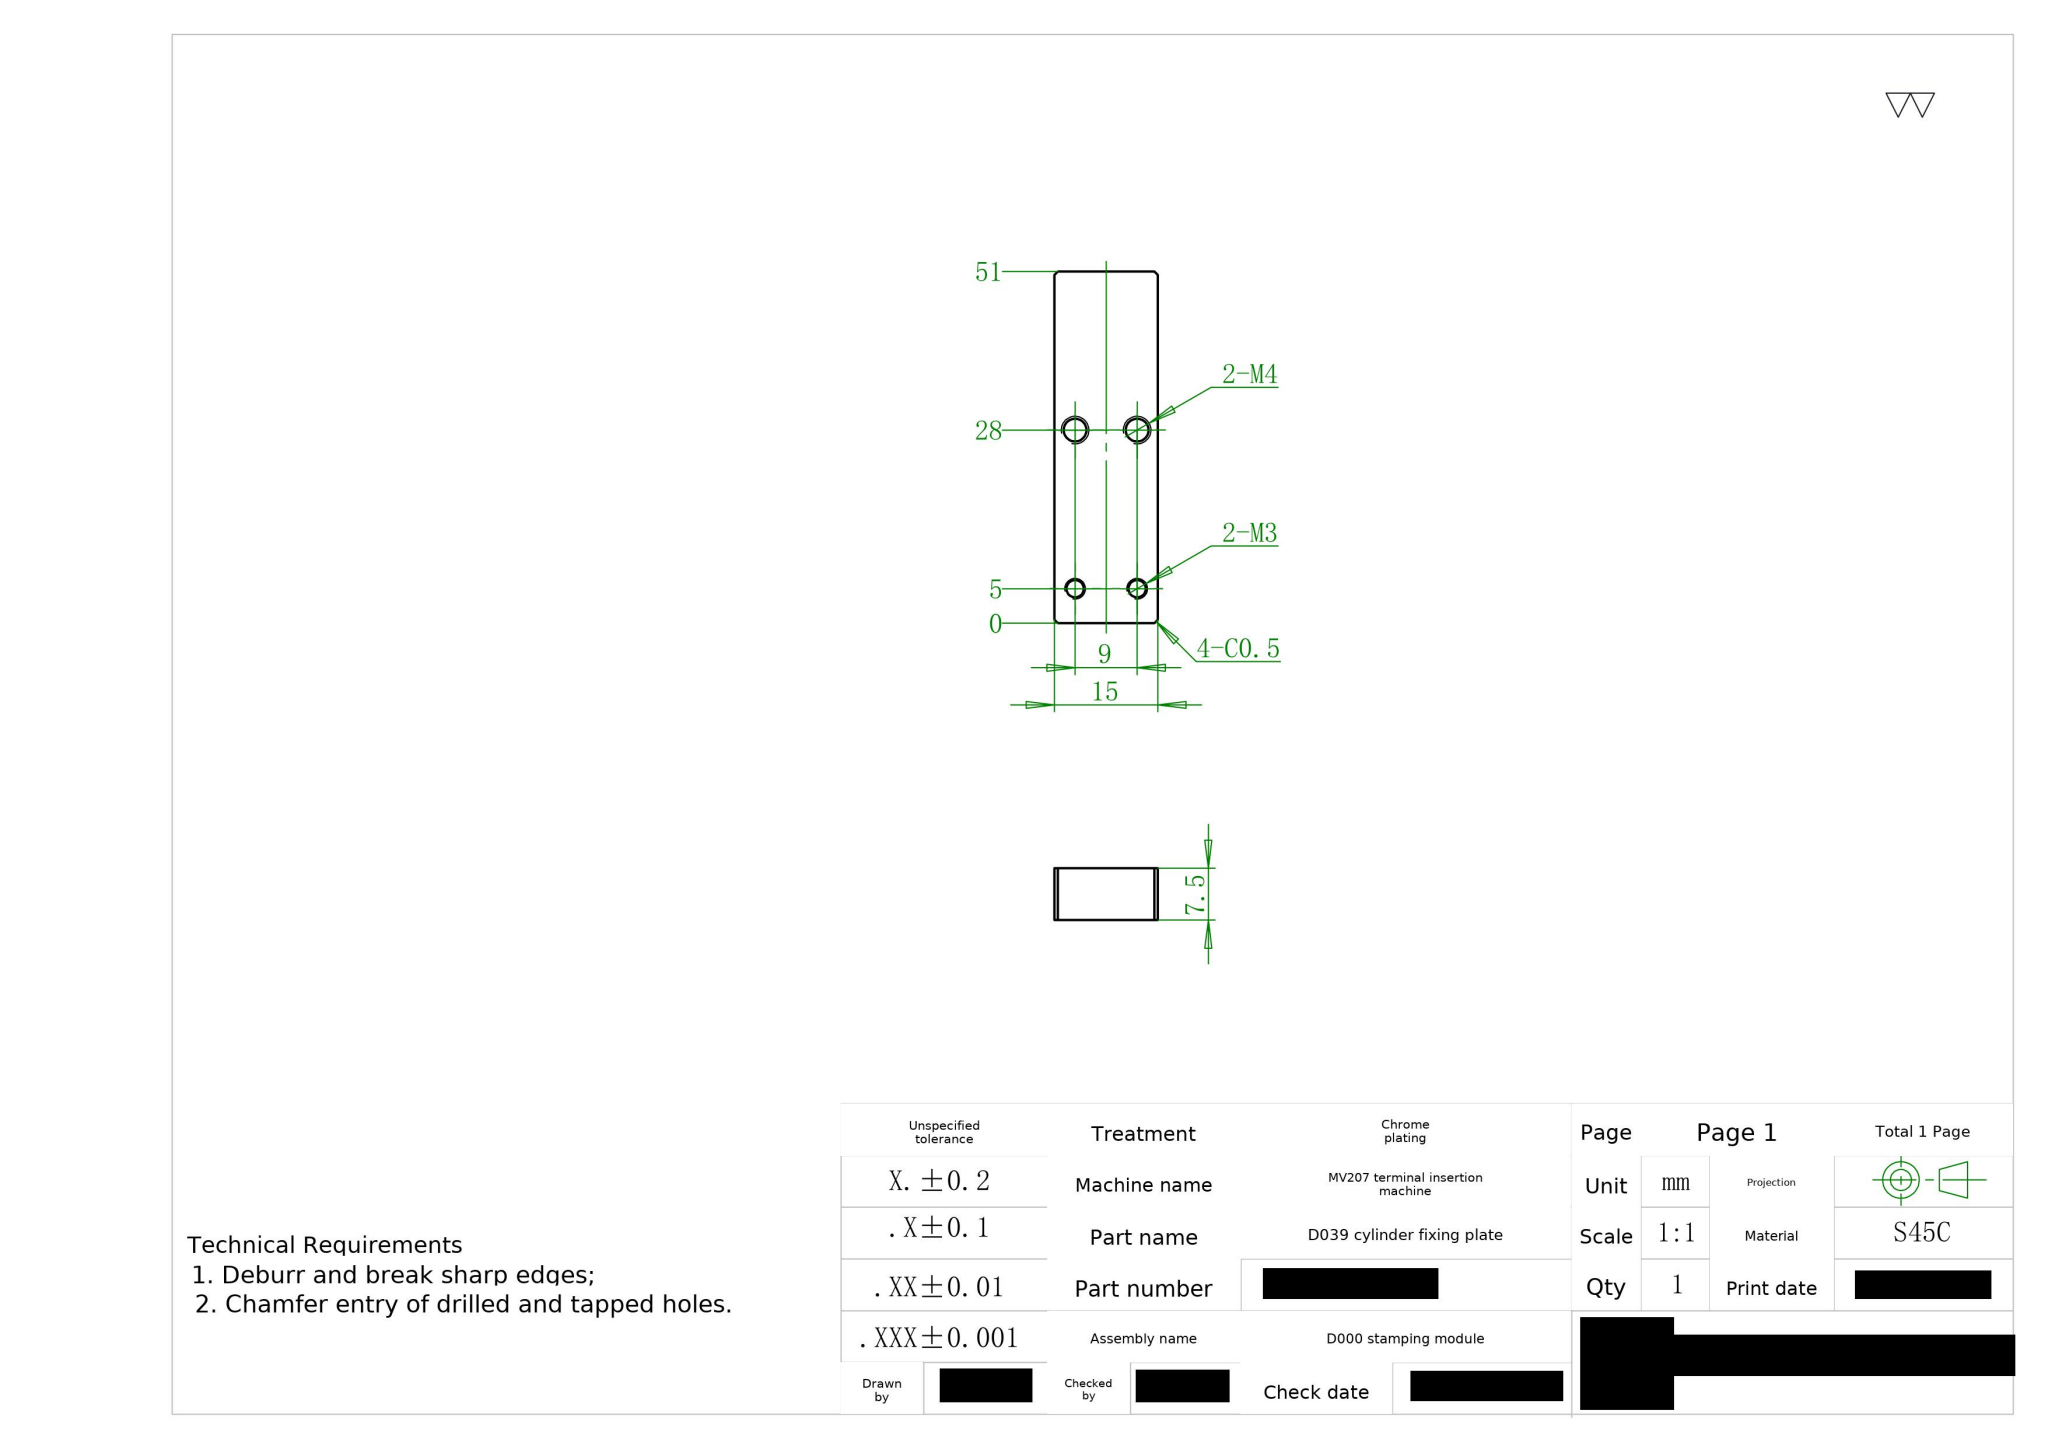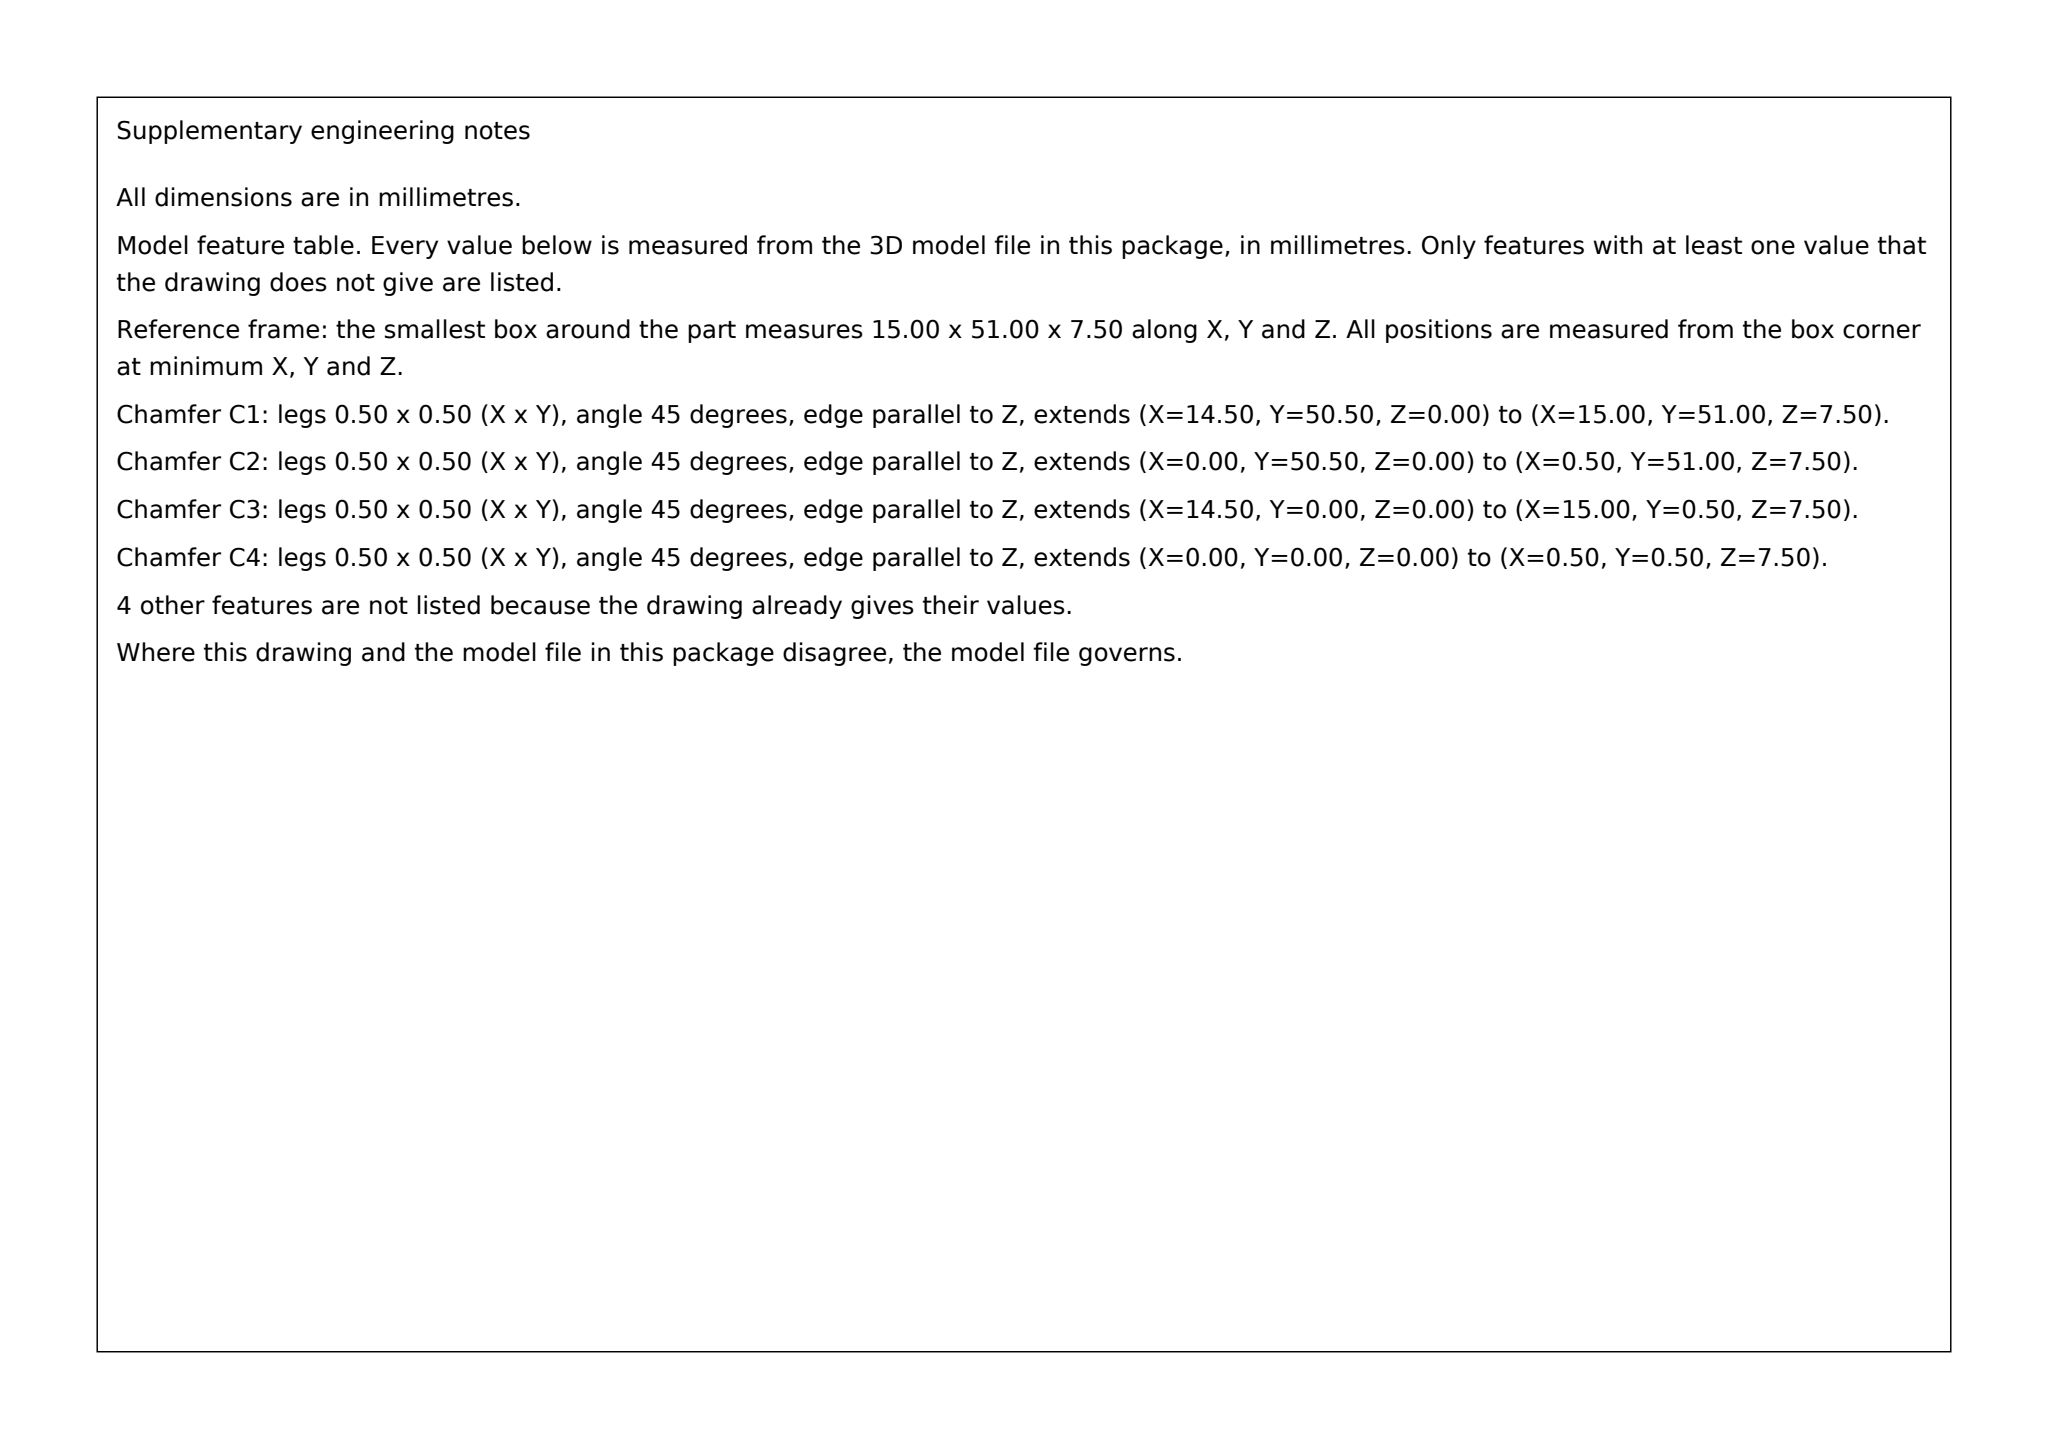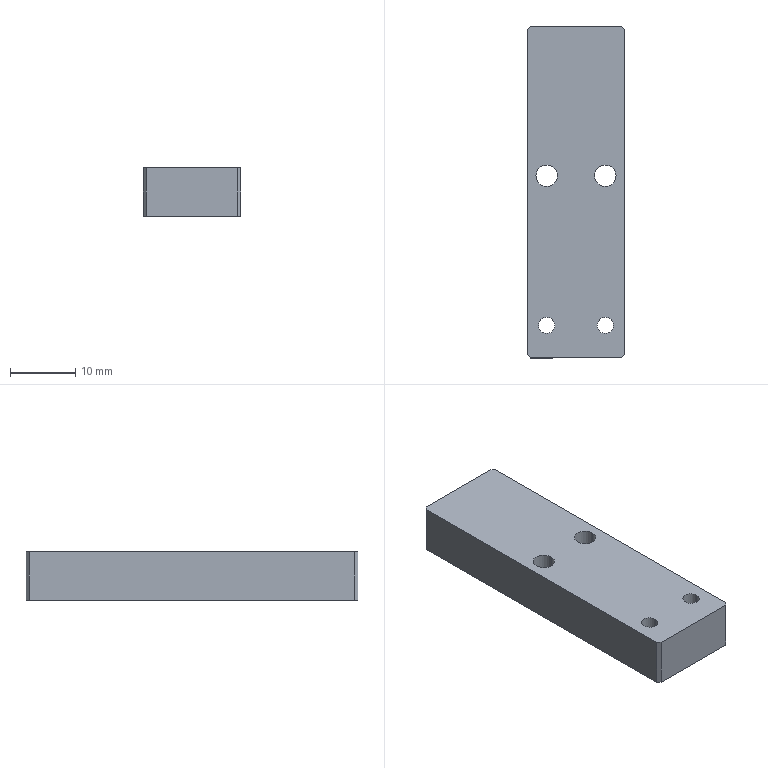Part | SolidWorks | mm | material S45C | 1 solid | 18 faces | box 15 x 51 x 7.5 mm | volume 5532 mm3 | plane 10 | cylinder 8 | commonest cylinder face diameters 2.5 x4 3.3 x4
build123d program:
from build123d import *

# Parameters (mm, degrees)
SKETCH1_W           = 15
SKETCH1_H           = 12
BOSS_EXTRUDE1_DEPTH = 25.52
SKETCH17_W          = 15
SKETCH17_H          = 7.5
BOSS_EXTRUDE2_DEPTH = 39
M4_TAPPED_HOLE1_D   = 3.3
SKETCH23_W          = 18.02
SKETCH23_H          = 12
CUT_EXTRUDE2_DEPTH  = 54.863
M3_TAPPED_HOLE3_D   = 2.5
CHAMFER1_SIZE       = 0.5


with BuildPart() as part:
    # Sketch1 → Boss-Extrude1 (new body)
    with BuildSketch(Plane.XY):
        Rectangle(SKETCH1_W, SKETCH1_H)
    extrude(amount=BOSS_EXTRUDE1_DEPTH)

    # Sketch17 → Boss-Extrude2 (add)
    with BuildSketch(Plane(origin=(0, 6, 0), x_dir=(1, 0, 0), z_dir=(0, 1, 0))):
        with Locations((0, -21.77)):
            Rectangle(SKETCH17_W, SKETCH17_H)
    extrude(amount=BOSS_EXTRUDE2_DEPTH)

    # M4 Tapped Hole1 (through all)
    with Locations(Plane.XY.offset(25.52)):
        with Locations((4.5, 22), (-4.5, 22)):
            Hole(M4_TAPPED_HOLE1_D / 2)

    # Sketch23 → Cut-Extrude2 (cut, through all)
    with BuildSketch(Plane.ZY.offset(7.5)):
        with Locations((9.01, 0)):
            Rectangle(SKETCH23_W, SKETCH23_H)
    extrude(amount=-CUT_EXTRUDE2_DEPTH, mode=Mode.SUBTRACT)

    # M3 Tapped Hole3 (through all)
    with Locations(Plane(origin=(0, 0, 18.02), x_dir=(-1, 0, 0), z_dir=(0, 0, -1))):
        with Locations((4.5, -1), (-4.5, -1)):
            Hole(M3_TAPPED_HOLE3_D / 2)

    # Chamfer1
    chamfer1_edges = [part.edges().sort_by_distance(p)[0] for p in [
        (7.5, 45, 21.77),
        (-7.5, 45, 21.77),
        (7.5, -6, 21.77),
        (-7.5, -6, 21.77),
    ]]
    chamfer(chamfer1_edges, length=CHAMFER1_SIZE)


solid = part.part
STEP:
#1=CARTESIAN_POINT('',(-3.25,-1.,25.52));
#2=VERTEX_POINT('',#1);
#3=CARTESIAN_POINT('',(-5.75,-1.,25.52));
#4=VERTEX_POINT('',#3);
#5=CARTESIAN_POINT('',(-4.5,-1.,25.52));
#6=DIRECTION('',(0.,0.,-1.));
#7=DIRECTION('',(-1.,0.,0.));
#8=AXIS2_PLACEMENT_3D('',#5,#6,#7);
#9=CIRCLE('',#8,1.25);
#10=EDGE_CURVE('',#2,#4,#9,.T.);
#11=ORIENTED_EDGE('',*,*,#10,.F.);
#12=CARTESIAN_POINT('',(-3.25,-1.,18.02));
#13=VERTEX_POINT('',#12);
#14=CARTESIAN_POINT('',(-3.25,-1.,18.02));
#15=DIRECTION('',(0.,0.,-1.));
#16=VECTOR('',#15,1000.);
#17=LINE('',#14,#16);
#18=EDGE_CURVE('',#2,#13,#17,.T.);
#19=ORIENTED_EDGE('',*,*,#18,.T.);
#20=CARTESIAN_POINT('',(-5.75,-1.,18.02));
#21=VERTEX_POINT('',#20);
#22=CARTESIAN_POINT('',(-4.5,-1.,18.02));
#23=DIRECTION('',(0.,0.,-1.));
#24=DIRECTION('',(-1.,0.,0.));
#25=AXIS2_PLACEMENT_3D('',#22,#23,#24);
#26=CIRCLE('',#25,1.25);
#27=EDGE_CURVE('',#13,#21,#26,.T.);
#28=ORIENTED_EDGE('',*,*,#27,.T.);
#29=CARTESIAN_POINT('',(-5.75,-1.,18.02));
#30=DIRECTION('',(0.,0.,-1.));
#31=VECTOR('',#30,1000.);
#32=LINE('',#29,#31);
#33=EDGE_CURVE('',#4,#21,#32,.T.);
#34=ORIENTED_EDGE('',*,*,#33,.F.);
#35=EDGE_LOOP('',(#11,#19,#28,#34));
#36=FACE_OUTER_BOUND('',#35,.T.);
#37=CARTESIAN_POINT('',(-4.5,-1.,18.02));
#38=DIRECTION('',(0.,0.,-1.));
#39=DIRECTION('',(-1.,0.,0.));
#40=AXIS2_PLACEMENT_3D('',#37,#38,#39);
#41=CYLINDRICAL_SURFACE('',#40,1.25);
#42=ADVANCED_FACE('',(#36),#41,.F.);
#43=CARTESIAN_POINT('',(5.75,-1.,25.52));
#44=VERTEX_POINT('',#43);
#45=CARTESIAN_POINT('',(3.25,-1.,25.52));
#46=VERTEX_POINT('',#45);
#47=CARTESIAN_POINT('',(4.5,-1.,25.52));
#48=DIRECTION('',(0.,0.,-1.));
#49=DIRECTION('',(-1.,0.,0.));
#50=AXIS2_PLACEMENT_3D('',#47,#48,#49);
#51=CIRCLE('',#50,1.25);
#52=EDGE_CURVE('',#44,#46,#51,.T.);
#53=ORIENTED_EDGE('',*,*,#52,.F.);
#54=CARTESIAN_POINT('',(5.75,-1.,18.02));
#55=VERTEX_POINT('',#54);
#56=CARTESIAN_POINT('',(5.75,-1.,18.02));
#57=DIRECTION('',(0.,0.,-1.));
#58=VECTOR('',#57,1000.);
#59=LINE('',#56,#58);
#60=EDGE_CURVE('',#44,#55,#59,.T.);
#61=ORIENTED_EDGE('',*,*,#60,.T.);
#62=CARTESIAN_POINT('',(3.25,-1.,18.02));
#63=VERTEX_POINT('',#62);
#64=CARTESIAN_POINT('',(4.5,-1.,18.02));
#65=DIRECTION('',(0.,0.,-1.));
#66=DIRECTION('',(-1.,0.,0.));
#67=AXIS2_PLACEMENT_3D('',#64,#65,#66);
#68=CIRCLE('',#67,1.25);
#69=EDGE_CURVE('',#55,#63,#68,.T.);
#70=ORIENTED_EDGE('',*,*,#69,.T.);
#71=CARTESIAN_POINT('',(3.25,-1.,18.02));
#72=DIRECTION('',(0.,0.,-1.));
#73=VECTOR('',#72,1000.);
#74=LINE('',#71,#73);
#75=EDGE_CURVE('',#46,#63,#74,.T.);
#76=ORIENTED_EDGE('',*,*,#75,.F.);
#77=EDGE_LOOP('',(#53,#61,#70,#76));
#78=FACE_OUTER_BOUND('',#77,.T.);
#79=CARTESIAN_POINT('',(4.5,-1.,18.02));
#80=DIRECTION('',(0.,0.,-1.));
#81=DIRECTION('',(-1.,0.,0.));
#82=AXIS2_PLACEMENT_3D('',#79,#80,#81);
#83=CYLINDRICAL_SURFACE('',#82,1.25);
#84=ADVANCED_FACE('',(#78),#83,.F.);
#85=CARTESIAN_POINT('',(2.85,22.,18.02));
#86=VERTEX_POINT('',#85);
#87=CARTESIAN_POINT('',(6.15,22.,18.02));
#88=VERTEX_POINT('',#87);
#89=CARTESIAN_POINT('',(4.5,22.,18.02));
#90=DIRECTION('',(0.,0.,1.));
#91=DIRECTION('',(1.,0.,0.));
#92=AXIS2_PLACEMENT_3D('',#89,#90,#91);
#93=CIRCLE('',#92,1.65);
#94=EDGE_CURVE('',#86,#88,#93,.T.);
#95=ORIENTED_EDGE('',*,*,#94,.F.);
#96=CARTESIAN_POINT('',(2.85,22.,25.52));
#97=VERTEX_POINT('',#96);
#98=CARTESIAN_POINT('',(2.85,22.,25.52));
#99=DIRECTION('',(0.,0.,1.));
#100=VECTOR('',#99,1000.);
#101=LINE('',#98,#100);
#102=EDGE_CURVE('',#86,#97,#101,.T.);
#103=ORIENTED_EDGE('',*,*,#102,.T.);
#104=CARTESIAN_POINT('',(6.15,22.,25.52));
#105=VERTEX_POINT('',#104);
#106=CARTESIAN_POINT('',(4.5,22.,25.52));
#107=DIRECTION('',(0.,0.,1.));
#108=DIRECTION('',(1.,0.,0.));
#109=AXIS2_PLACEMENT_3D('',#106,#107,#108);
#110=CIRCLE('',#109,1.65);
#111=EDGE_CURVE('',#97,#105,#110,.T.);
#112=ORIENTED_EDGE('',*,*,#111,.T.);
#113=CARTESIAN_POINT('',(6.15,22.,25.52));
#114=DIRECTION('',(0.,0.,1.));
#115=VECTOR('',#114,1000.);
#116=LINE('',#113,#115);
#117=EDGE_CURVE('',#88,#105,#116,.T.);
#118=ORIENTED_EDGE('',*,*,#117,.F.);
#119=EDGE_LOOP('',(#95,#103,#112,#118));
#120=FACE_OUTER_BOUND('',#119,.T.);
#121=CARTESIAN_POINT('',(4.5,22.,25.52));
#122=DIRECTION('',(0.,0.,1.));
#123=DIRECTION('',(1.,0.,0.));
#124=AXIS2_PLACEMENT_3D('',#121,#122,#123);
#125=CYLINDRICAL_SURFACE('',#124,1.65);
#126=ADVANCED_FACE('',(#120),#125,.F.);
#127=CARTESIAN_POINT('',(-6.15,22.,18.02));
#128=VERTEX_POINT('',#127);
#129=CARTESIAN_POINT('',(-2.85,22.,18.02));
#130=VERTEX_POINT('',#129);
#131=CARTESIAN_POINT('',(-4.5,22.,18.02));
#132=DIRECTION('',(0.,0.,1.));
#133=DIRECTION('',(1.,0.,0.));
#134=AXIS2_PLACEMENT_3D('',#131,#132,#133);
#135=CIRCLE('',#134,1.65);
#136=EDGE_CURVE('',#128,#130,#135,.T.);
#137=ORIENTED_EDGE('',*,*,#136,.F.);
#138=CARTESIAN_POINT('',(-6.15,22.,25.52));
#139=VERTEX_POINT('',#138);
#140=CARTESIAN_POINT('',(-6.15,22.,25.52));
#141=DIRECTION('',(0.,0.,1.));
#142=VECTOR('',#141,1000.);
#143=LINE('',#140,#142);
#144=EDGE_CURVE('',#128,#139,#143,.T.);
#145=ORIENTED_EDGE('',*,*,#144,.T.);
#146=CARTESIAN_POINT('',(-2.85,22.,25.52));
#147=VERTEX_POINT('',#146);
#148=CARTESIAN_POINT('',(-4.5,22.,25.52));
#149=DIRECTION('',(0.,0.,1.));
#150=DIRECTION('',(1.,0.,0.));
#151=AXIS2_PLACEMENT_3D('',#148,#149,#150);
#152=CIRCLE('',#151,1.65);
#153=EDGE_CURVE('',#139,#147,#152,.T.);
#154=ORIENTED_EDGE('',*,*,#153,.T.);
#155=CARTESIAN_POINT('',(-2.85,22.,25.52));
#156=DIRECTION('',(0.,0.,1.));
#157=VECTOR('',#156,1000.);
#158=LINE('',#155,#157);
#159=EDGE_CURVE('',#130,#147,#158,.T.);
#160=ORIENTED_EDGE('',*,*,#159,.F.);
#161=EDGE_LOOP('',(#137,#145,#154,#160));
#162=FACE_OUTER_BOUND('',#161,.T.);
#163=CARTESIAN_POINT('',(-4.5,22.,25.52));
#164=DIRECTION('',(0.,0.,1.));
#165=DIRECTION('',(1.,0.,0.));
#166=AXIS2_PLACEMENT_3D('',#163,#164,#165);
#167=CYLINDRICAL_SURFACE('',#166,1.65);
#168=ADVANCED_FACE('',(#162),#167,.F.);
#169=CARTESIAN_POINT('',(7.5,44.5,18.02));
#170=VERTEX_POINT('',#169);
#171=CARTESIAN_POINT('',(7.5,-5.5,18.02));
#172=VERTEX_POINT('',#171);
#173=CARTESIAN_POINT('',(7.5,45.,18.02));
#174=DIRECTION('',(0.,-1.,0.));
#175=VECTOR('',#174,1000.);
#176=LINE('',#173,#175);
#177=EDGE_CURVE('',#170,#172,#176,.T.);
#178=ORIENTED_EDGE('',*,*,#177,.F.);
#179=CARTESIAN_POINT('',(7.5,44.5,25.52));
#180=VERTEX_POINT('',#179);
#181=CARTESIAN_POINT('',(7.5,44.5,25.52));
#182=DIRECTION('',(0.,0.,1.));
#183=VECTOR('',#182,1000.);
#184=LINE('',#181,#183);
#185=EDGE_CURVE('',#170,#180,#184,.T.);
#186=ORIENTED_EDGE('',*,*,#185,.T.);
#187=CARTESIAN_POINT('',(7.5,-5.5,25.52));
#188=VERTEX_POINT('',#187);
#189=CARTESIAN_POINT('',(7.5,6.,25.52));
#190=DIRECTION('',(-0.,1.,0.));
#191=VECTOR('',#190,1000.);
#192=LINE('',#189,#191);
#193=EDGE_CURVE('',#188,#180,#192,.T.);
#194=ORIENTED_EDGE('',*,*,#193,.F.);
#195=CARTESIAN_POINT('',(7.5,-5.5,25.52));
#196=DIRECTION('',(0.,0.,-1.));
#197=VECTOR('',#196,1000.);
#198=LINE('',#195,#197);
#199=EDGE_CURVE('',#188,#172,#198,.T.);
#200=ORIENTED_EDGE('',*,*,#199,.T.);
#201=EDGE_LOOP('',(#178,#186,#194,#200));
#202=FACE_OUTER_BOUND('',#201,.T.);
#203=CARTESIAN_POINT('',(7.5,6.,25.52));
#204=DIRECTION('',(-1.,-0.,0.));
#205=DIRECTION('',(0.,-1.,0.));
#206=AXIS2_PLACEMENT_3D('',#203,#204,#205);
#207=PLANE('',#206);
#208=ADVANCED_FACE('',(#202),#207,.F.);
#209=CARTESIAN_POINT('',(-7.5,44.5,25.52));
#210=VERTEX_POINT('',#209);
#211=CARTESIAN_POINT('',(-7.5,-5.5,25.52));
#212=VERTEX_POINT('',#211);
#213=CARTESIAN_POINT('',(-7.5,6.,25.52));
#214=DIRECTION('',(0.,-1.,0.));
#215=VECTOR('',#214,1000.);
#216=LINE('',#213,#215);
#217=EDGE_CURVE('',#210,#212,#216,.T.);
#218=ORIENTED_EDGE('',*,*,#217,.F.);
#219=CARTESIAN_POINT('',(-7.5,44.5,18.02));
#220=VERTEX_POINT('',#219);
#221=CARTESIAN_POINT('',(-7.5,44.5,18.02));
#222=DIRECTION('',(0.,0.,-1.));
#223=VECTOR('',#222,1000.);
#224=LINE('',#221,#223);
#225=EDGE_CURVE('',#210,#220,#224,.T.);
#226=ORIENTED_EDGE('',*,*,#225,.T.);
#227=CARTESIAN_POINT('',(-7.5,-5.5,18.02));
#228=VERTEX_POINT('',#227);
#229=CARTESIAN_POINT('',(-7.5,45.,18.02));
#230=DIRECTION('',(0.,-1.,0.));
#231=VECTOR('',#230,1000.);
#232=LINE('',#229,#231);
#233=EDGE_CURVE('',#220,#228,#232,.T.);
#234=ORIENTED_EDGE('',*,*,#233,.T.);
#235=CARTESIAN_POINT('',(-7.5,-5.5,25.52));
#236=DIRECTION('',(0.,0.,1.));
#237=VECTOR('',#236,1000.);
#238=LINE('',#235,#237);
#239=EDGE_CURVE('',#228,#212,#238,.T.);
#240=ORIENTED_EDGE('',*,*,#239,.T.);
#241=EDGE_LOOP('',(#218,#226,#234,#240));
#242=FACE_OUTER_BOUND('',#241,.T.);
#243=CARTESIAN_POINT('',(-7.5,6.,25.52));
#244=DIRECTION('',(1.,0.,0.));
#245=DIRECTION('',(-0.,1.,0.));
#246=AXIS2_PLACEMENT_3D('',#243,#244,#245);
#247=PLANE('',#246);
#248=ADVANCED_FACE('',(#242),#247,.F.);
#249=CARTESIAN_POINT('',(7.,-6.,18.02));
#250=VERTEX_POINT('',#249);
#251=CARTESIAN_POINT('',(-7.,-6.,18.02));
#252=VERTEX_POINT('',#251);
#253=CARTESIAN_POINT('',(7.5,-6.,18.02));
#254=DIRECTION('',(-1.,-0.,0.));
#255=VECTOR('',#254,1000.);
#256=LINE('',#253,#255);
#257=EDGE_CURVE('',#250,#252,#256,.T.);
#258=ORIENTED_EDGE('',*,*,#257,.F.);
#259=CARTESIAN_POINT('',(7.,-6.,25.52));
#260=VERTEX_POINT('',#259);
#261=CARTESIAN_POINT('',(7.,-6.,25.52));
#262=DIRECTION('',(0.,0.,1.));
#263=VECTOR('',#262,1000.);
#264=LINE('',#261,#263);
#265=EDGE_CURVE('',#250,#260,#264,.T.);
#266=ORIENTED_EDGE('',*,*,#265,.T.);
#267=CARTESIAN_POINT('',(-7.,-6.,25.52));
#268=VERTEX_POINT('',#267);
#269=CARTESIAN_POINT('',(-7.5,-6.,25.52));
#270=DIRECTION('',(1.,0.,0.));
#271=VECTOR('',#270,1000.);
#272=LINE('',#269,#271);
#273=EDGE_CURVE('',#268,#260,#272,.T.);
#274=ORIENTED_EDGE('',*,*,#273,.F.);
#275=CARTESIAN_POINT('',(-7.,-6.,25.52));
#276=DIRECTION('',(0.,0.,-1.));
#277=VECTOR('',#276,1000.);
#278=LINE('',#275,#277);
#279=EDGE_CURVE('',#268,#252,#278,.T.);
#280=ORIENTED_EDGE('',*,*,#279,.T.);
#281=EDGE_LOOP('',(#258,#266,#274,#280));
#282=FACE_OUTER_BOUND('',#281,.T.);
#283=CARTESIAN_POINT('',(-7.5,-6.,25.52));
#284=DIRECTION('',(0.,1.,0.));
#285=DIRECTION('',(0.,0.,1.));
#286=AXIS2_PLACEMENT_3D('',#283,#284,#285);
#287=PLANE('',#286);
#288=ADVANCED_FACE('',(#282),#287,.F.);
#289=CARTESIAN_POINT('',(-4.5,-1.,25.52));
#290=DIRECTION('',(0.,0.,-1.));
#291=DIRECTION('',(-1.,0.,0.));
#292=AXIS2_PLACEMENT_3D('',#289,#290,#291);
#293=CIRCLE('',#292,1.25);
#294=EDGE_CURVE('',#4,#2,#293,.T.);
#295=ORIENTED_EDGE('',*,*,#294,.T.);
#296=ORIENTED_EDGE('',*,*,#10,.T.);
#297=EDGE_LOOP('',(#295,#296));
#298=FACE_BOUND('',#297,.T.);
#299=CARTESIAN_POINT('',(4.5,-1.,25.52));
#300=DIRECTION('',(0.,0.,-1.));
#301=DIRECTION('',(-1.,0.,0.));
#302=AXIS2_PLACEMENT_3D('',#299,#300,#301);
#303=CIRCLE('',#302,1.25);
#304=EDGE_CURVE('',#46,#44,#303,.T.);
#305=ORIENTED_EDGE('',*,*,#304,.T.);
#306=ORIENTED_EDGE('',*,*,#52,.T.);
#307=EDGE_LOOP('',(#305,#306));
#308=FACE_BOUND('',#307,.T.);
#309=CARTESIAN_POINT('',(4.5,22.,25.52));
#310=DIRECTION('',(0.,0.,1.));
#311=DIRECTION('',(1.,0.,0.));
#312=AXIS2_PLACEMENT_3D('',#309,#310,#311);
#313=CIRCLE('',#312,1.65);
#314=EDGE_CURVE('',#105,#97,#313,.T.);
#315=ORIENTED_EDGE('',*,*,#314,.F.);
#316=ORIENTED_EDGE('',*,*,#111,.F.);
#317=EDGE_LOOP('',(#315,#316));
#318=FACE_BOUND('',#317,.T.);
#319=CARTESIAN_POINT('',(-4.5,22.,25.52));
#320=DIRECTION('',(0.,0.,1.));
#321=DIRECTION('',(1.,0.,0.));
#322=AXIS2_PLACEMENT_3D('',#319,#320,#321);
#323=CIRCLE('',#322,1.65);
#324=EDGE_CURVE('',#147,#139,#323,.T.);
#325=ORIENTED_EDGE('',*,*,#324,.F.);
#326=ORIENTED_EDGE('',*,*,#153,.F.);
#327=EDGE_LOOP('',(#325,#326));
#328=FACE_BOUND('',#327,.T.);
#329=ORIENTED_EDGE('',*,*,#193,.T.);
#330=CARTESIAN_POINT('',(7.,45.,25.52));
#331=VERTEX_POINT('',#330);
#332=CARTESIAN_POINT('',(26.,26.,25.52));
#333=DIRECTION('',(-0.7071,0.7071,0.));
#334=VECTOR('',#333,1000.);
#335=LINE('',#332,#334);
#336=EDGE_CURVE('',#180,#331,#335,.T.);
#337=ORIENTED_EDGE('',*,*,#336,.T.);
#338=CARTESIAN_POINT('',(-7.,45.,25.52));
#339=VERTEX_POINT('',#338);
#340=CARTESIAN_POINT('',(7.5,45.,25.52));
#341=DIRECTION('',(1.,0.,-0.));
#342=VECTOR('',#341,1000.);
#343=LINE('',#340,#342);
#344=EDGE_CURVE('',#339,#331,#343,.T.);
#345=ORIENTED_EDGE('',*,*,#344,.F.);
#346=CARTESIAN_POINT('',(-26.,26.,25.52));
#347=DIRECTION('',(-0.7071,-0.7071,0.));
#348=VECTOR('',#347,1000.);
#349=LINE('',#346,#348);
#350=EDGE_CURVE('',#339,#210,#349,.T.);
#351=ORIENTED_EDGE('',*,*,#350,.T.);
#352=ORIENTED_EDGE('',*,*,#217,.T.);
#353=CARTESIAN_POINT('',(-6.5,-6.5,25.52));
#354=DIRECTION('',(0.7071,-0.7071,0.));
#355=VECTOR('',#354,1000.);
#356=LINE('',#353,#355);
#357=EDGE_CURVE('',#212,#268,#356,.T.);
#358=ORIENTED_EDGE('',*,*,#357,.T.);
#359=ORIENTED_EDGE('',*,*,#273,.T.);
#360=CARTESIAN_POINT('',(6.5,-6.5,25.52));
#361=DIRECTION('',(0.7071,0.7071,0.));
#362=VECTOR('',#361,1000.);
#363=LINE('',#360,#362);
#364=EDGE_CURVE('',#260,#188,#363,.T.);
#365=ORIENTED_EDGE('',*,*,#364,.T.);
#366=EDGE_LOOP('',(#329,#337,#345,#351,#352,#358,#359,#365));
#367=FACE_OUTER_BOUND('',#366,.T.);
#368=CARTESIAN_POINT('',(0.,0.,25.52));
#369=DIRECTION('',(0.,0.,1.));
#370=DIRECTION('',(1.,0.,0.));
#371=AXIS2_PLACEMENT_3D('',#368,#369,#370);
#372=PLANE('',#371);
#373=ADVANCED_FACE('',(#298,#308,#318,#328,#367),#372,.T.);
#374=CARTESIAN_POINT('',(-4.5,-1.,18.02));
#375=DIRECTION('',(0.,0.,-1.));
#376=DIRECTION('',(-1.,0.,0.));
#377=AXIS2_PLACEMENT_3D('',#374,#375,#376);
#378=CIRCLE('',#377,1.25);
#379=EDGE_CURVE('',#21,#13,#378,.T.);
#380=ORIENTED_EDGE('',*,*,#379,.F.);
#381=ORIENTED_EDGE('',*,*,#27,.F.);
#382=EDGE_LOOP('',(#380,#381));
#383=FACE_BOUND('',#382,.T.);
#384=CARTESIAN_POINT('',(4.5,-1.,18.02));
#385=DIRECTION('',(0.,0.,-1.));
#386=DIRECTION('',(-1.,0.,0.));
#387=AXIS2_PLACEMENT_3D('',#384,#385,#386);
#388=CIRCLE('',#387,1.25);
#389=EDGE_CURVE('',#63,#55,#388,.T.);
#390=ORIENTED_EDGE('',*,*,#389,.F.);
#391=ORIENTED_EDGE('',*,*,#69,.F.);
#392=EDGE_LOOP('',(#390,#391));
#393=FACE_BOUND('',#392,.T.);
#394=CARTESIAN_POINT('',(4.5,22.,18.02));
#395=DIRECTION('',(0.,0.,1.));
#396=DIRECTION('',(1.,0.,0.));
#397=AXIS2_PLACEMENT_3D('',#394,#395,#396);
#398=CIRCLE('',#397,1.65);
#399=EDGE_CURVE('',#88,#86,#398,.T.);
#400=ORIENTED_EDGE('',*,*,#399,.T.);
#401=ORIENTED_EDGE('',*,*,#94,.T.);
#402=EDGE_LOOP('',(#400,#401));
#403=FACE_BOUND('',#402,.T.);
#404=CARTESIAN_POINT('',(-4.5,22.,18.02));
#405=DIRECTION('',(0.,0.,1.));
#406=DIRECTION('',(1.,0.,0.));
#407=AXIS2_PLACEMENT_3D('',#404,#405,#406);
#408=CIRCLE('',#407,1.65);
#409=EDGE_CURVE('',#130,#128,#408,.T.);
#410=ORIENTED_EDGE('',*,*,#409,.T.);
#411=ORIENTED_EDGE('',*,*,#136,.T.);
#412=EDGE_LOOP('',(#410,#411));
#413=FACE_BOUND('',#412,.T.);
#414=CARTESIAN_POINT('',(7.,45.,18.02));
#415=VERTEX_POINT('',#414);
#416=CARTESIAN_POINT('',(-7.,45.,18.02));
#417=VERTEX_POINT('',#416);
#418=CARTESIAN_POINT('',(7.5,45.,18.02));
#419=DIRECTION('',(-1.,0.,0.));
#420=VECTOR('',#419,1000.);
#421=LINE('',#418,#420);
#422=EDGE_CURVE('',#415,#417,#421,.T.);
#423=ORIENTED_EDGE('',*,*,#422,.F.);
#424=CARTESIAN_POINT('',(7.,45.,18.02));
#425=DIRECTION('',(0.7071,-0.7071,0.));
#426=VECTOR('',#425,1000.);
#427=LINE('',#424,#426);
#428=EDGE_CURVE('',#415,#170,#427,.T.);
#429=ORIENTED_EDGE('',*,*,#428,.T.);
#430=ORIENTED_EDGE('',*,*,#177,.T.);
#431=CARTESIAN_POINT('',(7.5,-5.5,18.02));
#432=DIRECTION('',(-0.7071,-0.7071,0.));
#433=VECTOR('',#432,1000.);
#434=LINE('',#431,#433);
#435=EDGE_CURVE('',#172,#250,#434,.T.);
#436=ORIENTED_EDGE('',*,*,#435,.T.);
#437=ORIENTED_EDGE('',*,*,#257,.T.);
#438=CARTESIAN_POINT('',(-7.,-6.,18.02));
#439=DIRECTION('',(-0.7071,0.7071,0.));
#440=VECTOR('',#439,1000.);
#441=LINE('',#438,#440);
#442=EDGE_CURVE('',#252,#228,#441,.T.);
#443=ORIENTED_EDGE('',*,*,#442,.T.);
#444=ORIENTED_EDGE('',*,*,#233,.F.);
#445=CARTESIAN_POINT('',(-7.,45.,18.02));
#446=DIRECTION('',(0.7071,0.7071,0.));
#447=VECTOR('',#446,1000.);
#448=LINE('',#445,#447);
#449=EDGE_CURVE('',#220,#417,#448,.T.);
#450=ORIENTED_EDGE('',*,*,#449,.T.);
#451=EDGE_LOOP('',(#423,#429,#430,#436,#437,#443,#444,#450));
#452=FACE_OUTER_BOUND('',#451,.T.);
#453=CARTESIAN_POINT('',(7.5,45.,18.02));
#454=DIRECTION('',(0.,0.,1.));
#455=DIRECTION('',(1.,0.,0.));
#456=AXIS2_PLACEMENT_3D('',#453,#454,#455);
#457=PLANE('',#456);
#458=ADVANCED_FACE('',(#383,#393,#403,#413,#452),#457,.F.);
#459=ORIENTED_EDGE('',*,*,#344,.T.);
#460=CARTESIAN_POINT('',(7.,45.,18.02));
#461=DIRECTION('',(0.,0.,-1.));
#462=VECTOR('',#461,1000.);
#463=LINE('',#460,#462);
#464=EDGE_CURVE('',#331,#415,#463,.T.);
#465=ORIENTED_EDGE('',*,*,#464,.T.);
#466=ORIENTED_EDGE('',*,*,#422,.T.);
#467=CARTESIAN_POINT('',(-7.,45.,25.52));
#468=DIRECTION('',(0.,0.,1.));
#469=VECTOR('',#468,1000.);
#470=LINE('',#467,#469);
#471=EDGE_CURVE('',#417,#339,#470,.T.);
#472=ORIENTED_EDGE('',*,*,#471,.T.);
#473=EDGE_LOOP('',(#459,#465,#466,#472));
#474=FACE_OUTER_BOUND('',#473,.T.);
#475=CARTESIAN_POINT('',(0.,45.,0.));
#476=DIRECTION('',(0.,1.,0.));
#477=DIRECTION('',(0.,0.,1.));
#478=AXIS2_PLACEMENT_3D('',#475,#476,#477);
#479=PLANE('',#478);
#480=ADVANCED_FACE('',(#474),#479,.T.);
#481=ORIENTED_EDGE('',*,*,#144,.F.);
#482=ORIENTED_EDGE('',*,*,#409,.F.);
#483=ORIENTED_EDGE('',*,*,#159,.T.);
#484=ORIENTED_EDGE('',*,*,#324,.T.);
#485=EDGE_LOOP('',(#481,#482,#483,#484));
#486=FACE_OUTER_BOUND('',#485,.T.);
#487=CARTESIAN_POINT('',(-4.5,22.,25.52));
#488=DIRECTION('',(0.,0.,1.));
#489=DIRECTION('',(1.,0.,0.));
#490=AXIS2_PLACEMENT_3D('',#487,#488,#489);
#491=CYLINDRICAL_SURFACE('',#490,1.65);
#492=ADVANCED_FACE('',(#486),#491,.F.);
#493=ORIENTED_EDGE('',*,*,#102,.F.);
#494=ORIENTED_EDGE('',*,*,#399,.F.);
#495=ORIENTED_EDGE('',*,*,#117,.T.);
#496=ORIENTED_EDGE('',*,*,#314,.T.);
#497=EDGE_LOOP('',(#493,#494,#495,#496));
#498=FACE_OUTER_BOUND('',#497,.T.);
#499=CARTESIAN_POINT('',(4.5,22.,25.52));
#500=DIRECTION('',(0.,0.,1.));
#501=DIRECTION('',(1.,0.,0.));
#502=AXIS2_PLACEMENT_3D('',#499,#500,#501);
#503=CYLINDRICAL_SURFACE('',#502,1.65);
#504=ADVANCED_FACE('',(#498),#503,.F.);
#505=ORIENTED_EDGE('',*,*,#60,.F.);
#506=ORIENTED_EDGE('',*,*,#304,.F.);
#507=ORIENTED_EDGE('',*,*,#75,.T.);
#508=ORIENTED_EDGE('',*,*,#389,.T.);
#509=EDGE_LOOP('',(#505,#506,#507,#508));
#510=FACE_OUTER_BOUND('',#509,.T.);
#511=CARTESIAN_POINT('',(4.5,-1.,18.02));
#512=DIRECTION('',(0.,0.,-1.));
#513=DIRECTION('',(-1.,0.,0.));
#514=AXIS2_PLACEMENT_3D('',#511,#512,#513);
#515=CYLINDRICAL_SURFACE('',#514,1.25);
#516=ADVANCED_FACE('',(#510),#515,.F.);
#517=ORIENTED_EDGE('',*,*,#18,.F.);
#518=ORIENTED_EDGE('',*,*,#294,.F.);
#519=ORIENTED_EDGE('',*,*,#33,.T.);
#520=ORIENTED_EDGE('',*,*,#379,.T.);
#521=EDGE_LOOP('',(#517,#518,#519,#520));
#522=FACE_OUTER_BOUND('',#521,.T.);
#523=CARTESIAN_POINT('',(-4.5,-1.,18.02));
#524=DIRECTION('',(0.,0.,-1.));
#525=DIRECTION('',(-1.,0.,0.));
#526=AXIS2_PLACEMENT_3D('',#523,#524,#525);
#527=CYLINDRICAL_SURFACE('',#526,1.25);
#528=ADVANCED_FACE('',(#522),#527,.F.);
#529=ORIENTED_EDGE('',*,*,#336,.F.);
#530=ORIENTED_EDGE('',*,*,#185,.F.);
#531=ORIENTED_EDGE('',*,*,#428,.F.);
#532=ORIENTED_EDGE('',*,*,#464,.F.);
#533=EDGE_LOOP('',(#529,#530,#531,#532));
#534=FACE_OUTER_BOUND('',#533,.T.);
#535=CARTESIAN_POINT('',(7.,45.,0.));
#536=DIRECTION('',(0.7071,0.7071,0.));
#537=DIRECTION('',(0.,0.,1.));
#538=AXIS2_PLACEMENT_3D('',#535,#536,#537);
#539=PLANE('',#538);
#540=ADVANCED_FACE('',(#534),#539,.T.);
#541=ORIENTED_EDGE('',*,*,#449,.F.);
#542=ORIENTED_EDGE('',*,*,#225,.F.);
#543=ORIENTED_EDGE('',*,*,#350,.F.);
#544=ORIENTED_EDGE('',*,*,#471,.F.);
#545=EDGE_LOOP('',(#541,#542,#543,#544));
#546=FACE_OUTER_BOUND('',#545,.T.);
#547=CARTESIAN_POINT('',(-7.,45.,0.));
#548=DIRECTION('',(-0.7071,0.7071,0.));
#549=DIRECTION('',(0.,0.,-1.));
#550=AXIS2_PLACEMENT_3D('',#547,#548,#549);
#551=PLANE('',#550);
#552=ADVANCED_FACE('',(#546),#551,.T.);
#553=ORIENTED_EDGE('',*,*,#364,.F.);
#554=ORIENTED_EDGE('',*,*,#265,.F.);
#555=ORIENTED_EDGE('',*,*,#435,.F.);
#556=ORIENTED_EDGE('',*,*,#199,.F.);
#557=EDGE_LOOP('',(#553,#554,#555,#556));
#558=FACE_OUTER_BOUND('',#557,.T.);
#559=CARTESIAN_POINT('',(7.5,-5.5,25.52));
#560=DIRECTION('',(-0.7071,0.7071,0.));
#561=DIRECTION('',(0.,0.,-1.));
#562=AXIS2_PLACEMENT_3D('',#559,#560,#561);
#563=PLANE('',#562);
#564=ADVANCED_FACE('',(#558),#563,.F.);
#565=ORIENTED_EDGE('',*,*,#357,.F.);
#566=ORIENTED_EDGE('',*,*,#239,.F.);
#567=ORIENTED_EDGE('',*,*,#442,.F.);
#568=ORIENTED_EDGE('',*,*,#279,.F.);
#569=EDGE_LOOP('',(#565,#566,#567,#568));
#570=FACE_OUTER_BOUND('',#569,.T.);
#571=CARTESIAN_POINT('',(-7.,-6.,25.52));
#572=DIRECTION('',(0.7071,0.7071,0.));
#573=DIRECTION('',(0.,0.,-1.));
#574=AXIS2_PLACEMENT_3D('',#571,#572,#573);
#575=PLANE('',#574);
#576=ADVANCED_FACE('',(#570),#575,.F.);
#577=CLOSED_SHELL('',(#42,#84,#126,#168,#208,#248,#288,#373,#458,#480,#492,#504,#516,#528,#540,#552,#564,#576));
#578=MANIFOLD_SOLID_BREP('',#577);
#579=CARTESIAN_POINT('',(0.,0.,0.));
#580=DIRECTION('',(0.,0.,1.));
#581=DIRECTION('',(1.,0.,0.));
#582=AXIS2_PLACEMENT_3D('',#579,#580,#581);
#583=(LENGTH_UNIT()NAMED_UNIT(*)SI_UNIT(.MILLI.,.METRE.));
#584=UNCERTAINTY_MEASURE_WITH_UNIT(LENGTH_MEASURE(0.00001),#583,'','');
#585=(NAMED_UNIT(*)PLANE_ANGLE_UNIT()SI_UNIT($,.RADIAN.));
#586=(NAMED_UNIT(*)SI_UNIT($,.STERADIAN.)SOLID_ANGLE_UNIT());
#587=(GEOMETRIC_REPRESENTATION_CONTEXT(3)GLOBAL_UNCERTAINTY_ASSIGNED_CONTEXT((#584))GLOBAL_UNIT_ASSIGNED_CONTEXT((#583,#585,#586))REPRESENTATION_CONTEXT('',''));
#588=ADVANCED_BREP_SHAPE_REPRESENTATION('',(#578,#582),#587);